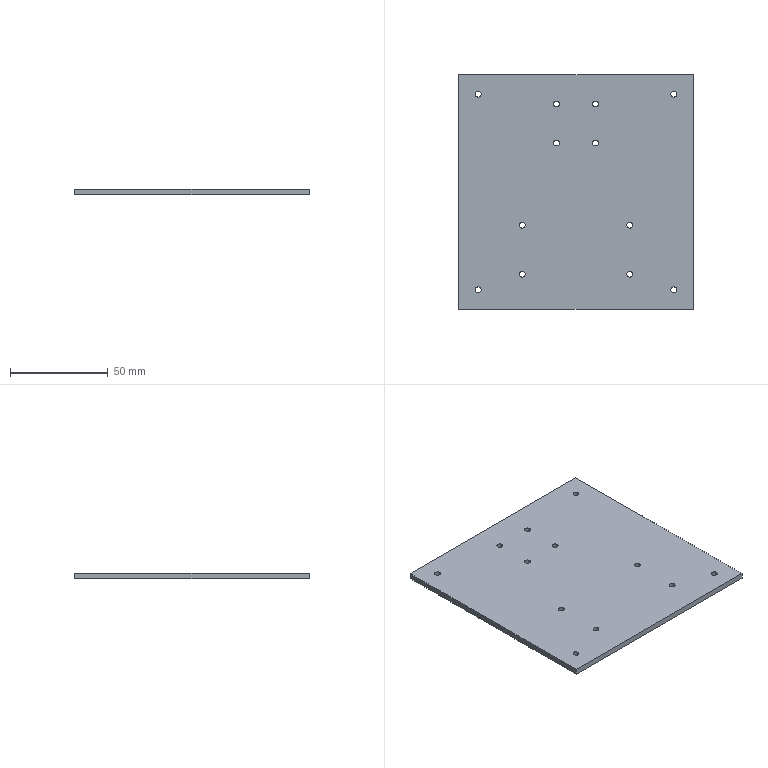Component | SolidWorks | Assembly3-1_Plate3-1 | 1 solid | 30 faces | box 120 x 120 x 3 mm | volume 42946 mm3 | cylinder 24 | plane 6 | commonest cylinder face diameters 3 x24
build123d program:
from build123d import *

# Parameters (mm, degrees)
SKETCH1_W           = 120
SKETCH1_H           = 120
BOSS_EXTRUDE1_DEPTH = 3
SKETCH2_R           = 1.5
CUT_EXTRUDE1_DEPTH  = 3
SKETCH5_R           = 1.5
CUT_EXTRUDE2_DEPTH  = 10


with BuildPart() as part:
    # Sketch1 → Boss-Extrude1 (new body)
    with BuildSketch(Plane.XY):
        Rectangle(SKETCH1_W, SKETCH1_H)
    extrude(amount=BOSS_EXTRUDE1_DEPTH)

    # Sketch2 → Cut-Extrude1 (cut)
    with BuildSketch(Plane.XY.offset(3)):
        with Locations((-50, 50)):
            Circle(SKETCH2_R)
        with Locations(Location((50, 50, 0), (0, 0, 180))):
            Circle(SKETCH2_R)
        with Locations((50, -50)):
            Circle(SKETCH2_R)
        with Locations(Location((-50, -50, 0), (0, 0, 180))):
            Circle(SKETCH2_R)
    extrude(amount=-CUT_EXTRUDE1_DEPTH, mode=Mode.SUBTRACT)

    # Sketch5 → Cut-Extrude2 (cut)
    with BuildSketch(Plane.XY.offset(3)):
        with Locations((-27.5, 42)):
            Circle(SKETCH5_R)
        with Locations((27.5, 42)):
            Circle(SKETCH5_R)
        with Locations((-10, -45)):
            Circle(SKETCH5_R)
        with Locations((10, -45)):
            Circle(SKETCH5_R)
        with Locations((-27.5, 17)):
            Circle(SKETCH5_R)
        with Locations((27.5, 17)):
            Circle(SKETCH5_R)
        with Locations((-10, -25)):
            Circle(SKETCH5_R)
        with Locations((10, -25)):
            Circle(SKETCH5_R)
    extrude(amount=-CUT_EXTRUDE2_DEPTH, mode=Mode.SUBTRACT)


solid = part.part

# Placed as in the assembly
solid = solid.moved(Location((0, 0, 52), (180, 0, 0)))
STEP:
#1=COLOUR_RGB('',0.7922,0.8196,0.9333);
#2=FILL_AREA_STYLE_COLOUR('',#1);
#3=FILL_AREA_STYLE('',(#2));
#4=SURFACE_STYLE_FILL_AREA(#3);
#5=SURFACE_SIDE_STYLE('',(#4));
#6=SURFACE_STYLE_USAGE(.BOTH.,#5);
#7=PRESENTATION_STYLE_ASSIGNMENT((#6));
#8=CARTESIAN_POINT('',(-1.142,-0.6693,2.047));
#9=VERTEX_POINT('',#8);
#10=CARTESIAN_POINT('',(-1.024,-0.6693,2.047));
#11=VERTEX_POINT('',#10);
#12=CARTESIAN_POINT('',(-1.083,-0.6693,2.047));
#13=DIRECTION('',(-0.,-0.,-1.));
#14=DIRECTION('',(1.,0.,0.));
#15=AXIS2_PLACEMENT_3D('',#12,#13,#14);
#16=CIRCLE('',#15,0.05906);
#17=EDGE_CURVE('',#9,#11,#16,.T.);
#18=ORIENTED_EDGE('',*,*,#17,.F.);
#19=CARTESIAN_POINT('',(-1.142,-0.6693,1.929));
#20=VERTEX_POINT('',#19);
#21=CARTESIAN_POINT('',(-1.142,-0.6693,2.323));
#22=DIRECTION('',(-0.,-0.,-1.));
#23=VECTOR('',#22,39.37);
#24=LINE('',#21,#23);
#25=EDGE_CURVE('',#9,#20,#24,.T.);
#26=ORIENTED_EDGE('',*,*,#25,.T.);
#27=CARTESIAN_POINT('',(-1.024,-0.6693,1.929));
#28=VERTEX_POINT('',#27);
#29=CARTESIAN_POINT('',(-1.083,-0.6693,1.929));
#30=DIRECTION('',(-0.,-0.,-1.));
#31=DIRECTION('',(1.,0.,0.));
#32=AXIS2_PLACEMENT_3D('',#29,#30,#31);
#33=CIRCLE('',#32,0.05906);
#34=EDGE_CURVE('',#20,#28,#33,.T.);
#35=ORIENTED_EDGE('',*,*,#34,.T.);
#36=CARTESIAN_POINT('',(-1.024,-0.6693,2.323));
#37=DIRECTION('',(-0.,-0.,-1.));
#38=VECTOR('',#37,39.37);
#39=LINE('',#36,#38);
#40=EDGE_CURVE('',#11,#28,#39,.T.);
#41=ORIENTED_EDGE('',*,*,#40,.F.);
#42=EDGE_LOOP('',(#18,#26,#35,#41));
#43=FACE_OUTER_BOUND('',#42,.T.);
#44=CARTESIAN_POINT('',(-1.083,-0.6693,2.323));
#45=DIRECTION('',(-0.,-0.,-1.));
#46=DIRECTION('',(1.,0.,0.));
#47=AXIS2_PLACEMENT_3D('',#44,#45,#46);
#48=CYLINDRICAL_SURFACE('',#47,0.05906);
#49=ADVANCED_FACE('',(#43),#48,.F.);
#50=CARTESIAN_POINT('',(0.3346,1.772,2.047));
#51=VERTEX_POINT('',#50);
#52=CARTESIAN_POINT('',(0.4528,1.772,2.047));
#53=VERTEX_POINT('',#52);
#54=CARTESIAN_POINT('',(0.3937,1.772,2.047));
#55=DIRECTION('',(-0.,-0.,-1.));
#56=DIRECTION('',(1.,0.,0.));
#57=AXIS2_PLACEMENT_3D('',#54,#55,#56);
#58=CIRCLE('',#57,0.05906);
#59=EDGE_CURVE('',#51,#53,#58,.T.);
#60=ORIENTED_EDGE('',*,*,#59,.F.);
#61=CARTESIAN_POINT('',(0.3346,1.772,1.929));
#62=VERTEX_POINT('',#61);
#63=CARTESIAN_POINT('',(0.3346,1.772,2.323));
#64=DIRECTION('',(-0.,-0.,-1.));
#65=VECTOR('',#64,39.37);
#66=LINE('',#63,#65);
#67=EDGE_CURVE('',#51,#62,#66,.T.);
#68=ORIENTED_EDGE('',*,*,#67,.T.);
#69=CARTESIAN_POINT('',(0.4528,1.772,1.929));
#70=VERTEX_POINT('',#69);
#71=CARTESIAN_POINT('',(0.3937,1.772,1.929));
#72=DIRECTION('',(-0.,-0.,-1.));
#73=DIRECTION('',(-1.,0.,0.));
#74=AXIS2_PLACEMENT_3D('',#71,#72,#73);
#75=CIRCLE('',#74,0.05906);
#76=EDGE_CURVE('',#62,#70,#75,.T.);
#77=ORIENTED_EDGE('',*,*,#76,.T.);
#78=CARTESIAN_POINT('',(0.4528,1.772,2.323));
#79=DIRECTION('',(-0.,-0.,-1.));
#80=VECTOR('',#79,39.37);
#81=LINE('',#78,#80);
#82=EDGE_CURVE('',#53,#70,#81,.T.);
#83=ORIENTED_EDGE('',*,*,#82,.F.);
#84=EDGE_LOOP('',(#60,#68,#77,#83));
#85=FACE_OUTER_BOUND('',#84,.T.);
#86=CARTESIAN_POINT('',(0.3937,1.772,2.323));
#87=DIRECTION('',(-0.,-0.,-1.));
#88=DIRECTION('',(1.,0.,0.));
#89=AXIS2_PLACEMENT_3D('',#86,#87,#88);
#90=CYLINDRICAL_SURFACE('',#89,0.05906);
#91=ADVANCED_FACE('',(#85),#90,.F.);
#92=CARTESIAN_POINT('',(-0.4528,1.772,2.047));
#93=VERTEX_POINT('',#92);
#94=CARTESIAN_POINT('',(-0.3346,1.772,2.047));
#95=VERTEX_POINT('',#94);
#96=CARTESIAN_POINT('',(-0.3937,1.772,2.047));
#97=DIRECTION('',(-0.,-0.,-1.));
#98=DIRECTION('',(1.,0.,0.));
#99=AXIS2_PLACEMENT_3D('',#96,#97,#98);
#100=CIRCLE('',#99,0.05906);
#101=EDGE_CURVE('',#93,#95,#100,.T.);
#102=ORIENTED_EDGE('',*,*,#101,.F.);
#103=CARTESIAN_POINT('',(-0.4528,1.772,1.929));
#104=VERTEX_POINT('',#103);
#105=CARTESIAN_POINT('',(-0.4528,1.772,2.323));
#106=DIRECTION('',(-0.,-0.,-1.));
#107=VECTOR('',#106,39.37);
#108=LINE('',#105,#107);
#109=EDGE_CURVE('',#93,#104,#108,.T.);
#110=ORIENTED_EDGE('',*,*,#109,.T.);
#111=CARTESIAN_POINT('',(-0.3346,1.772,1.929));
#112=VERTEX_POINT('',#111);
#113=CARTESIAN_POINT('',(-0.3937,1.772,1.929));
#114=DIRECTION('',(-0.,-0.,-1.));
#115=DIRECTION('',(1.,0.,0.));
#116=AXIS2_PLACEMENT_3D('',#113,#114,#115);
#117=CIRCLE('',#116,0.05906);
#118=EDGE_CURVE('',#104,#112,#117,.T.);
#119=ORIENTED_EDGE('',*,*,#118,.T.);
#120=CARTESIAN_POINT('',(-0.3346,1.772,2.323));
#121=DIRECTION('',(-0.,-0.,-1.));
#122=VECTOR('',#121,39.37);
#123=LINE('',#120,#122);
#124=EDGE_CURVE('',#95,#112,#123,.T.);
#125=ORIENTED_EDGE('',*,*,#124,.F.);
#126=EDGE_LOOP('',(#102,#110,#119,#125));
#127=FACE_OUTER_BOUND('',#126,.T.);
#128=CARTESIAN_POINT('',(-0.3937,1.772,2.323));
#129=DIRECTION('',(-0.,-0.,-1.));
#130=DIRECTION('',(1.,0.,0.));
#131=AXIS2_PLACEMENT_3D('',#128,#129,#130);
#132=CYLINDRICAL_SURFACE('',#131,0.05906);
#133=ADVANCED_FACE('',(#127),#132,.F.);
#134=CARTESIAN_POINT('',(1.024,-1.654,2.047));
#135=VERTEX_POINT('',#134);
#136=CARTESIAN_POINT('',(1.142,-1.654,2.047));
#137=VERTEX_POINT('',#136);
#138=CARTESIAN_POINT('',(1.083,-1.654,2.047));
#139=DIRECTION('',(-0.,-0.,-1.));
#140=DIRECTION('',(1.,0.,0.));
#141=AXIS2_PLACEMENT_3D('',#138,#139,#140);
#142=CIRCLE('',#141,0.05906);
#143=EDGE_CURVE('',#135,#137,#142,.T.);
#144=ORIENTED_EDGE('',*,*,#143,.F.);
#145=CARTESIAN_POINT('',(1.024,-1.654,1.929));
#146=VERTEX_POINT('',#145);
#147=CARTESIAN_POINT('',(1.024,-1.654,2.323));
#148=DIRECTION('',(-0.,-0.,-1.));
#149=VECTOR('',#148,39.37);
#150=LINE('',#147,#149);
#151=EDGE_CURVE('',#135,#146,#150,.T.);
#152=ORIENTED_EDGE('',*,*,#151,.T.);
#153=CARTESIAN_POINT('',(1.142,-1.654,1.929));
#154=VERTEX_POINT('',#153);
#155=CARTESIAN_POINT('',(1.083,-1.654,1.929));
#156=DIRECTION('',(-0.,-0.,-1.));
#157=DIRECTION('',(-1.,0.,0.));
#158=AXIS2_PLACEMENT_3D('',#155,#156,#157);
#159=CIRCLE('',#158,0.05906);
#160=EDGE_CURVE('',#146,#154,#159,.T.);
#161=ORIENTED_EDGE('',*,*,#160,.T.);
#162=CARTESIAN_POINT('',(1.142,-1.654,2.323));
#163=DIRECTION('',(-0.,-0.,-1.));
#164=VECTOR('',#163,39.37);
#165=LINE('',#162,#164);
#166=EDGE_CURVE('',#137,#154,#165,.T.);
#167=ORIENTED_EDGE('',*,*,#166,.F.);
#168=EDGE_LOOP('',(#144,#152,#161,#167));
#169=FACE_OUTER_BOUND('',#168,.T.);
#170=CARTESIAN_POINT('',(1.083,-1.654,2.323));
#171=DIRECTION('',(-0.,-0.,-1.));
#172=DIRECTION('',(1.,0.,0.));
#173=AXIS2_PLACEMENT_3D('',#170,#171,#172);
#174=CYLINDRICAL_SURFACE('',#173,0.05906);
#175=ADVANCED_FACE('',(#169),#174,.F.);
#176=CARTESIAN_POINT('',(0.3346,0.9843,2.047));
#177=VERTEX_POINT('',#176);
#178=CARTESIAN_POINT('',(0.4528,0.9843,2.047));
#179=VERTEX_POINT('',#178);
#180=CARTESIAN_POINT('',(0.3937,0.9843,2.047));
#181=DIRECTION('',(-0.,-0.,-1.));
#182=DIRECTION('',(1.,0.,0.));
#183=AXIS2_PLACEMENT_3D('',#180,#181,#182);
#184=CIRCLE('',#183,0.05906);
#185=EDGE_CURVE('',#177,#179,#184,.T.);
#186=ORIENTED_EDGE('',*,*,#185,.F.);
#187=CARTESIAN_POINT('',(0.3346,0.9843,1.929));
#188=VERTEX_POINT('',#187);
#189=CARTESIAN_POINT('',(0.3346,0.9843,2.323));
#190=DIRECTION('',(-0.,-0.,-1.));
#191=VECTOR('',#190,39.37);
#192=LINE('',#189,#191);
#193=EDGE_CURVE('',#177,#188,#192,.T.);
#194=ORIENTED_EDGE('',*,*,#193,.T.);
#195=CARTESIAN_POINT('',(0.4528,0.9843,1.929));
#196=VERTEX_POINT('',#195);
#197=CARTESIAN_POINT('',(0.3937,0.9843,1.929));
#198=DIRECTION('',(-0.,-0.,-1.));
#199=DIRECTION('',(1.,0.,0.));
#200=AXIS2_PLACEMENT_3D('',#197,#198,#199);
#201=CIRCLE('',#200,0.05906);
#202=EDGE_CURVE('',#188,#196,#201,.T.);
#203=ORIENTED_EDGE('',*,*,#202,.T.);
#204=CARTESIAN_POINT('',(0.4528,0.9843,2.323));
#205=DIRECTION('',(-0.,-0.,-1.));
#206=VECTOR('',#205,39.37);
#207=LINE('',#204,#206);
#208=EDGE_CURVE('',#179,#196,#207,.T.);
#209=ORIENTED_EDGE('',*,*,#208,.F.);
#210=EDGE_LOOP('',(#186,#194,#203,#209));
#211=FACE_OUTER_BOUND('',#210,.T.);
#212=CARTESIAN_POINT('',(0.3937,0.9843,2.323));
#213=DIRECTION('',(-0.,-0.,-1.));
#214=DIRECTION('',(1.,0.,0.));
#215=AXIS2_PLACEMENT_3D('',#212,#213,#214);
#216=CYLINDRICAL_SURFACE('',#215,0.05906);
#217=ADVANCED_FACE('',(#211),#216,.F.);
#218=CARTESIAN_POINT('',(-0.4528,0.9843,2.047));
#219=VERTEX_POINT('',#218);
#220=CARTESIAN_POINT('',(-0.3346,0.9843,2.047));
#221=VERTEX_POINT('',#220);
#222=CARTESIAN_POINT('',(-0.3937,0.9843,2.047));
#223=DIRECTION('',(-0.,-0.,-1.));
#224=DIRECTION('',(1.,0.,0.));
#225=AXIS2_PLACEMENT_3D('',#222,#223,#224);
#226=CIRCLE('',#225,0.05906);
#227=EDGE_CURVE('',#219,#221,#226,.T.);
#228=ORIENTED_EDGE('',*,*,#227,.F.);
#229=CARTESIAN_POINT('',(-0.4528,0.9843,1.929));
#230=VERTEX_POINT('',#229);
#231=CARTESIAN_POINT('',(-0.4528,0.9843,2.323));
#232=DIRECTION('',(-0.,-0.,-1.));
#233=VECTOR('',#232,39.37);
#234=LINE('',#231,#233);
#235=EDGE_CURVE('',#219,#230,#234,.T.);
#236=ORIENTED_EDGE('',*,*,#235,.T.);
#237=CARTESIAN_POINT('',(-0.3346,0.9843,1.929));
#238=VERTEX_POINT('',#237);
#239=CARTESIAN_POINT('',(-0.3937,0.9843,1.929));
#240=DIRECTION('',(-0.,-0.,-1.));
#241=DIRECTION('',(1.,0.,0.));
#242=AXIS2_PLACEMENT_3D('',#239,#240,#241);
#243=CIRCLE('',#242,0.05906);
#244=EDGE_CURVE('',#230,#238,#243,.T.);
#245=ORIENTED_EDGE('',*,*,#244,.T.);
#246=CARTESIAN_POINT('',(-0.3346,0.9843,2.323));
#247=DIRECTION('',(-0.,-0.,-1.));
#248=VECTOR('',#247,39.37);
#249=LINE('',#246,#248);
#250=EDGE_CURVE('',#221,#238,#249,.T.);
#251=ORIENTED_EDGE('',*,*,#250,.F.);
#252=EDGE_LOOP('',(#228,#236,#245,#251));
#253=FACE_OUTER_BOUND('',#252,.T.);
#254=CARTESIAN_POINT('',(-0.3937,0.9843,2.323));
#255=DIRECTION('',(-0.,-0.,-1.));
#256=DIRECTION('',(1.,0.,0.));
#257=AXIS2_PLACEMENT_3D('',#254,#255,#256);
#258=CYLINDRICAL_SURFACE('',#257,0.05906);
#259=ADVANCED_FACE('',(#253),#258,.F.);
#260=CARTESIAN_POINT('',(1.024,-0.6693,2.047));
#261=VERTEX_POINT('',#260);
#262=CARTESIAN_POINT('',(1.142,-0.6693,2.047));
#263=VERTEX_POINT('',#262);
#264=CARTESIAN_POINT('',(1.083,-0.6693,2.047));
#265=DIRECTION('',(-0.,-0.,-1.));
#266=DIRECTION('',(1.,0.,0.));
#267=AXIS2_PLACEMENT_3D('',#264,#265,#266);
#268=CIRCLE('',#267,0.05906);
#269=EDGE_CURVE('',#261,#263,#268,.T.);
#270=ORIENTED_EDGE('',*,*,#269,.F.);
#271=CARTESIAN_POINT('',(1.024,-0.6693,1.929));
#272=VERTEX_POINT('',#271);
#273=CARTESIAN_POINT('',(1.024,-0.6693,2.323));
#274=DIRECTION('',(-0.,-0.,-1.));
#275=VECTOR('',#274,39.37);
#276=LINE('',#273,#275);
#277=EDGE_CURVE('',#261,#272,#276,.T.);
#278=ORIENTED_EDGE('',*,*,#277,.T.);
#279=CARTESIAN_POINT('',(1.142,-0.6693,1.929));
#280=VERTEX_POINT('',#279);
#281=CARTESIAN_POINT('',(1.083,-0.6693,1.929));
#282=DIRECTION('',(-0.,-0.,-1.));
#283=DIRECTION('',(-1.,0.,0.));
#284=AXIS2_PLACEMENT_3D('',#281,#282,#283);
#285=CIRCLE('',#284,0.05906);
#286=EDGE_CURVE('',#272,#280,#285,.T.);
#287=ORIENTED_EDGE('',*,*,#286,.T.);
#288=CARTESIAN_POINT('',(1.142,-0.6693,2.323));
#289=DIRECTION('',(-0.,-0.,-1.));
#290=VECTOR('',#289,39.37);
#291=LINE('',#288,#290);
#292=EDGE_CURVE('',#263,#280,#291,.T.);
#293=ORIENTED_EDGE('',*,*,#292,.F.);
#294=EDGE_LOOP('',(#270,#278,#287,#293));
#295=FACE_OUTER_BOUND('',#294,.T.);
#296=CARTESIAN_POINT('',(1.083,-0.6693,2.323));
#297=DIRECTION('',(-0.,-0.,-1.));
#298=DIRECTION('',(1.,0.,0.));
#299=AXIS2_PLACEMENT_3D('',#296,#297,#298);
#300=CYLINDRICAL_SURFACE('',#299,0.05906);
#301=ADVANCED_FACE('',(#295),#300,.F.);
#302=CARTESIAN_POINT('',(-1.142,-1.654,2.047));
#303=VERTEX_POINT('',#302);
#304=CARTESIAN_POINT('',(-1.024,-1.654,2.047));
#305=VERTEX_POINT('',#304);
#306=CARTESIAN_POINT('',(-1.083,-1.654,2.047));
#307=DIRECTION('',(-0.,-0.,-1.));
#308=DIRECTION('',(1.,0.,0.));
#309=AXIS2_PLACEMENT_3D('',#306,#307,#308);
#310=CIRCLE('',#309,0.05906);
#311=EDGE_CURVE('',#303,#305,#310,.T.);
#312=ORIENTED_EDGE('',*,*,#311,.F.);
#313=CARTESIAN_POINT('',(-1.142,-1.654,1.929));
#314=VERTEX_POINT('',#313);
#315=CARTESIAN_POINT('',(-1.142,-1.654,2.323));
#316=DIRECTION('',(-0.,-0.,-1.));
#317=VECTOR('',#316,39.37);
#318=LINE('',#315,#317);
#319=EDGE_CURVE('',#303,#314,#318,.T.);
#320=ORIENTED_EDGE('',*,*,#319,.T.);
#321=CARTESIAN_POINT('',(-1.024,-1.654,1.929));
#322=VERTEX_POINT('',#321);
#323=CARTESIAN_POINT('',(-1.083,-1.654,1.929));
#324=DIRECTION('',(-0.,-0.,-1.));
#325=DIRECTION('',(1.,0.,0.));
#326=AXIS2_PLACEMENT_3D('',#323,#324,#325);
#327=CIRCLE('',#326,0.05906);
#328=EDGE_CURVE('',#314,#322,#327,.T.);
#329=ORIENTED_EDGE('',*,*,#328,.T.);
#330=CARTESIAN_POINT('',(-1.024,-1.654,2.323));
#331=DIRECTION('',(-0.,-0.,-1.));
#332=VECTOR('',#331,39.37);
#333=LINE('',#330,#332);
#334=EDGE_CURVE('',#305,#322,#333,.T.);
#335=ORIENTED_EDGE('',*,*,#334,.F.);
#336=EDGE_LOOP('',(#312,#320,#329,#335));
#337=FACE_OUTER_BOUND('',#336,.T.);
#338=CARTESIAN_POINT('',(-1.083,-1.654,2.323));
#339=DIRECTION('',(-0.,-0.,-1.));
#340=DIRECTION('',(1.,0.,0.));
#341=AXIS2_PLACEMENT_3D('',#338,#339,#340);
#342=CYLINDRICAL_SURFACE('',#341,0.05906);
#343=ADVANCED_FACE('',(#337),#342,.F.);
#344=CARTESIAN_POINT('',(-2.028,1.969,2.047));
#345=VERTEX_POINT('',#344);
#346=CARTESIAN_POINT('',(-1.909,1.969,2.047));
#347=VERTEX_POINT('',#346);
#348=CARTESIAN_POINT('',(-1.969,1.969,2.047));
#349=DIRECTION('',(-0.,-0.,-1.));
#350=DIRECTION('',(-1.,0.,0.));
#351=AXIS2_PLACEMENT_3D('',#348,#349,#350);
#352=CIRCLE('',#351,0.05906);
#353=EDGE_CURVE('',#345,#347,#352,.T.);
#354=ORIENTED_EDGE('',*,*,#353,.F.);
#355=CARTESIAN_POINT('',(-2.028,1.969,1.929));
#356=VERTEX_POINT('',#355);
#357=CARTESIAN_POINT('',(-2.028,1.969,2.047));
#358=DIRECTION('',(-0.,-0.,-1.));
#359=VECTOR('',#358,39.37);
#360=LINE('',#357,#359);
#361=EDGE_CURVE('',#345,#356,#360,.T.);
#362=ORIENTED_EDGE('',*,*,#361,.T.);
#363=CARTESIAN_POINT('',(-1.909,1.969,1.929));
#364=VERTEX_POINT('',#363);
#365=CARTESIAN_POINT('',(-1.969,1.969,1.929));
#366=DIRECTION('',(-0.,-0.,-1.));
#367=DIRECTION('',(-1.,0.,0.));
#368=AXIS2_PLACEMENT_3D('',#365,#366,#367);
#369=CIRCLE('',#368,0.05906);
#370=EDGE_CURVE('',#356,#364,#369,.T.);
#371=ORIENTED_EDGE('',*,*,#370,.T.);
#372=CARTESIAN_POINT('',(-1.909,1.969,2.047));
#373=DIRECTION('',(-0.,-0.,-1.));
#374=VECTOR('',#373,39.37);
#375=LINE('',#372,#374);
#376=EDGE_CURVE('',#347,#364,#375,.T.);
#377=ORIENTED_EDGE('',*,*,#376,.F.);
#378=EDGE_LOOP('',(#354,#362,#371,#377));
#379=FACE_OUTER_BOUND('',#378,.T.);
#380=CARTESIAN_POINT('',(-1.969,1.969,2.047));
#381=DIRECTION('',(-0.,-0.,-1.));
#382=DIRECTION('',(1.,0.,0.));
#383=AXIS2_PLACEMENT_3D('',#380,#381,#382);
#384=CYLINDRICAL_SURFACE('',#383,0.05906);
#385=ADVANCED_FACE('',(#379),#384,.F.);
#386=CARTESIAN_POINT('',(1.909,1.969,2.047));
#387=VERTEX_POINT('',#386);
#388=CARTESIAN_POINT('',(2.028,1.969,2.047));
#389=VERTEX_POINT('',#388);
#390=CARTESIAN_POINT('',(1.969,1.969,2.047));
#391=DIRECTION('',(-0.,-0.,-1.));
#392=DIRECTION('',(1.,0.,0.));
#393=AXIS2_PLACEMENT_3D('',#390,#391,#392);
#394=CIRCLE('',#393,0.05906);
#395=EDGE_CURVE('',#387,#389,#394,.T.);
#396=ORIENTED_EDGE('',*,*,#395,.F.);
#397=CARTESIAN_POINT('',(1.909,1.969,1.929));
#398=VERTEX_POINT('',#397);
#399=CARTESIAN_POINT('',(1.909,1.969,2.047));
#400=DIRECTION('',(-0.,-0.,-1.));
#401=VECTOR('',#400,39.37);
#402=LINE('',#399,#401);
#403=EDGE_CURVE('',#387,#398,#402,.T.);
#404=ORIENTED_EDGE('',*,*,#403,.T.);
#405=CARTESIAN_POINT('',(2.028,1.969,1.929));
#406=VERTEX_POINT('',#405);
#407=CARTESIAN_POINT('',(1.969,1.969,1.929));
#408=DIRECTION('',(-0.,-0.,-1.));
#409=DIRECTION('',(1.,0.,0.));
#410=AXIS2_PLACEMENT_3D('',#407,#408,#409);
#411=CIRCLE('',#410,0.05906);
#412=EDGE_CURVE('',#398,#406,#411,.T.);
#413=ORIENTED_EDGE('',*,*,#412,.T.);
#414=CARTESIAN_POINT('',(2.028,1.969,2.047));
#415=DIRECTION('',(-0.,-0.,-1.));
#416=VECTOR('',#415,39.37);
#417=LINE('',#414,#416);
#418=EDGE_CURVE('',#389,#406,#417,.T.);
#419=ORIENTED_EDGE('',*,*,#418,.F.);
#420=EDGE_LOOP('',(#396,#404,#413,#419));
#421=FACE_OUTER_BOUND('',#420,.T.);
#422=CARTESIAN_POINT('',(1.969,1.969,2.047));
#423=DIRECTION('',(-0.,-0.,-1.));
#424=DIRECTION('',(1.,0.,0.));
#425=AXIS2_PLACEMENT_3D('',#422,#423,#424);
#426=CYLINDRICAL_SURFACE('',#425,0.05906);
#427=ADVANCED_FACE('',(#421),#426,.F.);
#428=CARTESIAN_POINT('',(1.909,-1.969,2.047));
#429=VERTEX_POINT('',#428);
#430=CARTESIAN_POINT('',(2.028,-1.969,2.047));
#431=VERTEX_POINT('',#430);
#432=CARTESIAN_POINT('',(1.969,-1.969,2.047));
#433=DIRECTION('',(-0.,-0.,-1.));
#434=DIRECTION('',(-1.,0.,0.));
#435=AXIS2_PLACEMENT_3D('',#432,#433,#434);
#436=CIRCLE('',#435,0.05906);
#437=EDGE_CURVE('',#429,#431,#436,.T.);
#438=ORIENTED_EDGE('',*,*,#437,.F.);
#439=CARTESIAN_POINT('',(1.909,-1.969,1.929));
#440=VERTEX_POINT('',#439);
#441=CARTESIAN_POINT('',(1.909,-1.969,2.047));
#442=DIRECTION('',(-0.,-0.,-1.));
#443=VECTOR('',#442,39.37);
#444=LINE('',#441,#443);
#445=EDGE_CURVE('',#429,#440,#444,.T.);
#446=ORIENTED_EDGE('',*,*,#445,.T.);
#447=CARTESIAN_POINT('',(2.028,-1.969,1.929));
#448=VERTEX_POINT('',#447);
#449=CARTESIAN_POINT('',(1.969,-1.969,1.929));
#450=DIRECTION('',(-0.,-0.,-1.));
#451=DIRECTION('',(-1.,0.,0.));
#452=AXIS2_PLACEMENT_3D('',#449,#450,#451);
#453=CIRCLE('',#452,0.05906);
#454=EDGE_CURVE('',#440,#448,#453,.T.);
#455=ORIENTED_EDGE('',*,*,#454,.T.);
#456=CARTESIAN_POINT('',(2.028,-1.969,2.047));
#457=DIRECTION('',(-0.,-0.,-1.));
#458=VECTOR('',#457,39.37);
#459=LINE('',#456,#458);
#460=EDGE_CURVE('',#431,#448,#459,.T.);
#461=ORIENTED_EDGE('',*,*,#460,.F.);
#462=EDGE_LOOP('',(#438,#446,#455,#461));
#463=FACE_OUTER_BOUND('',#462,.T.);
#464=CARTESIAN_POINT('',(1.969,-1.969,2.047));
#465=DIRECTION('',(-0.,-0.,-1.));
#466=DIRECTION('',(1.,0.,0.));
#467=AXIS2_PLACEMENT_3D('',#464,#465,#466);
#468=CYLINDRICAL_SURFACE('',#467,0.05906);
#469=ADVANCED_FACE('',(#463),#468,.F.);
#470=CARTESIAN_POINT('',(-2.028,-1.969,2.047));
#471=VERTEX_POINT('',#470);
#472=CARTESIAN_POINT('',(-1.909,-1.969,2.047));
#473=VERTEX_POINT('',#472);
#474=CARTESIAN_POINT('',(-1.969,-1.969,2.047));
#475=DIRECTION('',(-0.,-0.,-1.));
#476=DIRECTION('',(1.,0.,0.));
#477=AXIS2_PLACEMENT_3D('',#474,#475,#476);
#478=CIRCLE('',#477,0.05906);
#479=EDGE_CURVE('',#471,#473,#478,.T.);
#480=ORIENTED_EDGE('',*,*,#479,.F.);
#481=CARTESIAN_POINT('',(-2.028,-1.969,1.929));
#482=VERTEX_POINT('',#481);
#483=CARTESIAN_POINT('',(-2.028,-1.969,2.047));
#484=DIRECTION('',(-0.,-0.,-1.));
#485=VECTOR('',#484,39.37);
#486=LINE('',#483,#485);
#487=EDGE_CURVE('',#471,#482,#486,.T.);
#488=ORIENTED_EDGE('',*,*,#487,.T.);
#489=CARTESIAN_POINT('',(-1.909,-1.969,1.929));
#490=VERTEX_POINT('',#489);
#491=CARTESIAN_POINT('',(-1.969,-1.969,1.929));
#492=DIRECTION('',(-0.,-0.,-1.));
#493=DIRECTION('',(1.,0.,0.));
#494=AXIS2_PLACEMENT_3D('',#491,#492,#493);
#495=CIRCLE('',#494,0.05906);
#496=EDGE_CURVE('',#482,#490,#495,.T.);
#497=ORIENTED_EDGE('',*,*,#496,.T.);
#498=CARTESIAN_POINT('',(-1.909,-1.969,2.047));
#499=DIRECTION('',(-0.,-0.,-1.));
#500=VECTOR('',#499,39.37);
#501=LINE('',#498,#500);
#502=EDGE_CURVE('',#473,#490,#501,.T.);
#503=ORIENTED_EDGE('',*,*,#502,.F.);
#504=EDGE_LOOP('',(#480,#488,#497,#503));
#505=FACE_OUTER_BOUND('',#504,.T.);
#506=CARTESIAN_POINT('',(-1.969,-1.969,2.047));
#507=DIRECTION('',(-0.,-0.,-1.));
#508=DIRECTION('',(1.,0.,0.));
#509=AXIS2_PLACEMENT_3D('',#506,#507,#508);
#510=CYLINDRICAL_SURFACE('',#509,0.05906);
#511=ADVANCED_FACE('',(#505),#510,.F.);
#512=CARTESIAN_POINT('',(2.362,2.362,2.047));
#513=VERTEX_POINT('',#512);
#514=CARTESIAN_POINT('',(2.362,-2.362,2.047));
#515=VERTEX_POINT('',#514);
#516=CARTESIAN_POINT('',(2.362,-2.362,2.047));
#517=DIRECTION('',(0.,-1.,0.));
#518=VECTOR('',#517,39.37);
#519=LINE('',#516,#518);
#520=EDGE_CURVE('',#513,#515,#519,.T.);
#521=ORIENTED_EDGE('',*,*,#520,.T.);
#522=CARTESIAN_POINT('',(2.362,-2.362,1.929));
#523=VERTEX_POINT('',#522);
#524=CARTESIAN_POINT('',(2.362,-2.362,1.929));
#525=DIRECTION('',(0.,0.,1.));
#526=VECTOR('',#525,39.37);
#527=LINE('',#524,#526);
#528=EDGE_CURVE('',#523,#515,#527,.T.);
#529=ORIENTED_EDGE('',*,*,#528,.F.);
#530=CARTESIAN_POINT('',(2.362,2.362,1.929));
#531=VERTEX_POINT('',#530);
#532=CARTESIAN_POINT('',(2.362,-2.362,1.929));
#533=DIRECTION('',(0.,-1.,0.));
#534=VECTOR('',#533,39.37);
#535=LINE('',#532,#534);
#536=EDGE_CURVE('',#531,#523,#535,.T.);
#537=ORIENTED_EDGE('',*,*,#536,.F.);
#538=CARTESIAN_POINT('',(2.362,2.362,1.929));
#539=DIRECTION('',(0.,0.,1.));
#540=VECTOR('',#539,39.37);
#541=LINE('',#538,#540);
#542=EDGE_CURVE('',#531,#513,#541,.T.);
#543=ORIENTED_EDGE('',*,*,#542,.T.);
#544=EDGE_LOOP('',(#521,#529,#537,#543));
#545=FACE_OUTER_BOUND('',#544,.T.);
#546=CARTESIAN_POINT('',(2.362,-2.362,1.929));
#547=DIRECTION('',(-1.,-0.,0.));
#548=DIRECTION('',(-0.,1.,-0.));
#549=AXIS2_PLACEMENT_3D('',#546,#547,#548);
#550=PLANE('',#549);
#551=ADVANCED_FACE('',(#545),#550,.F.);
#552=CARTESIAN_POINT('',(-2.362,-2.362,2.047));
#553=VERTEX_POINT('',#552);
#554=CARTESIAN_POINT('',(-2.362,-2.362,2.047));
#555=DIRECTION('',(-1.,-0.,0.));
#556=VECTOR('',#555,39.37);
#557=LINE('',#554,#556);
#558=EDGE_CURVE('',#515,#553,#557,.T.);
#559=ORIENTED_EDGE('',*,*,#558,.T.);
#560=CARTESIAN_POINT('',(-2.362,-2.362,1.929));
#561=VERTEX_POINT('',#560);
#562=CARTESIAN_POINT('',(-2.362,-2.362,1.929));
#563=DIRECTION('',(0.,0.,1.));
#564=VECTOR('',#563,39.37);
#565=LINE('',#562,#564);
#566=EDGE_CURVE('',#561,#553,#565,.T.);
#567=ORIENTED_EDGE('',*,*,#566,.F.);
#568=CARTESIAN_POINT('',(-2.362,-2.362,1.929));
#569=DIRECTION('',(-1.,-0.,0.));
#570=VECTOR('',#569,39.37);
#571=LINE('',#568,#570);
#572=EDGE_CURVE('',#523,#561,#571,.T.);
#573=ORIENTED_EDGE('',*,*,#572,.F.);
#574=ORIENTED_EDGE('',*,*,#528,.T.);
#575=EDGE_LOOP('',(#559,#567,#573,#574));
#576=FACE_OUTER_BOUND('',#575,.T.);
#577=CARTESIAN_POINT('',(-2.362,-2.362,1.929));
#578=DIRECTION('',(-0.,1.,-0.));
#579=DIRECTION('',(0.,0.,1.));
#580=AXIS2_PLACEMENT_3D('',#577,#578,#579);
#581=PLANE('',#580);
#582=ADVANCED_FACE('',(#576),#581,.F.);
#583=CARTESIAN_POINT('',(-2.362,2.362,2.047));
#584=VERTEX_POINT('',#583);
#585=CARTESIAN_POINT('',(-2.362,-2.362,2.047));
#586=DIRECTION('',(-0.,1.,-0.));
#587=VECTOR('',#586,39.37);
#588=LINE('',#585,#587);
#589=EDGE_CURVE('',#553,#584,#588,.T.);
#590=ORIENTED_EDGE('',*,*,#589,.T.);
#591=CARTESIAN_POINT('',(-2.362,2.362,1.929));
#592=VERTEX_POINT('',#591);
#593=CARTESIAN_POINT('',(-2.362,2.362,1.929));
#594=DIRECTION('',(0.,0.,1.));
#595=VECTOR('',#594,39.37);
#596=LINE('',#593,#595);
#597=EDGE_CURVE('',#592,#584,#596,.T.);
#598=ORIENTED_EDGE('',*,*,#597,.F.);
#599=CARTESIAN_POINT('',(-2.362,-2.362,1.929));
#600=DIRECTION('',(-0.,1.,-0.));
#601=VECTOR('',#600,39.37);
#602=LINE('',#599,#601);
#603=EDGE_CURVE('',#561,#592,#602,.T.);
#604=ORIENTED_EDGE('',*,*,#603,.F.);
#605=ORIENTED_EDGE('',*,*,#566,.T.);
#606=EDGE_LOOP('',(#590,#598,#604,#605));
#607=FACE_OUTER_BOUND('',#606,.T.);
#608=CARTESIAN_POINT('',(-2.362,-2.362,1.929));
#609=DIRECTION('',(1.,0.,-0.));
#610=DIRECTION('',(0.,-1.,0.));
#611=AXIS2_PLACEMENT_3D('',#608,#609,#610);
#612=PLANE('',#611);
#613=ADVANCED_FACE('',(#607),#612,.F.);
#614=CARTESIAN_POINT('',(-2.362,2.362,2.047));
#615=DIRECTION('',(1.,0.,-0.));
#616=VECTOR('',#615,39.37);
#617=LINE('',#614,#616);
#618=EDGE_CURVE('',#584,#513,#617,.T.);
#619=ORIENTED_EDGE('',*,*,#618,.T.);
#620=ORIENTED_EDGE('',*,*,#542,.F.);
#621=CARTESIAN_POINT('',(-2.362,2.362,1.929));
#622=DIRECTION('',(1.,0.,-0.));
#623=VECTOR('',#622,39.37);
#624=LINE('',#621,#623);
#625=EDGE_CURVE('',#592,#531,#624,.T.);
#626=ORIENTED_EDGE('',*,*,#625,.F.);
#627=ORIENTED_EDGE('',*,*,#597,.T.);
#628=EDGE_LOOP('',(#619,#620,#626,#627));
#629=FACE_OUTER_BOUND('',#628,.T.);
#630=CARTESIAN_POINT('',(-2.362,2.362,1.929));
#631=DIRECTION('',(0.,-1.,0.));
#632=DIRECTION('',(-0.,-0.,-1.));
#633=AXIS2_PLACEMENT_3D('',#630,#631,#632);
#634=PLANE('',#633);
#635=ADVANCED_FACE('',(#629),#634,.F.);
#636=CARTESIAN_POINT('',(-1.083,-0.6693,1.929));
#637=DIRECTION('',(-0.,-0.,-1.));
#638=DIRECTION('',(1.,0.,0.));
#639=AXIS2_PLACEMENT_3D('',#636,#637,#638);
#640=CIRCLE('',#639,0.05906);
#641=EDGE_CURVE('',#28,#20,#640,.T.);
#642=ORIENTED_EDGE('',*,*,#641,.F.);
#643=ORIENTED_EDGE('',*,*,#34,.F.);
#644=EDGE_LOOP('',(#642,#643));
#645=FACE_BOUND('',#644,.T.);
#646=CARTESIAN_POINT('',(0.3937,1.772,1.929));
#647=DIRECTION('',(-0.,-0.,-1.));
#648=DIRECTION('',(-1.,0.,0.));
#649=AXIS2_PLACEMENT_3D('',#646,#647,#648);
#650=CIRCLE('',#649,0.05906);
#651=EDGE_CURVE('',#70,#62,#650,.T.);
#652=ORIENTED_EDGE('',*,*,#651,.F.);
#653=ORIENTED_EDGE('',*,*,#76,.F.);
#654=EDGE_LOOP('',(#652,#653));
#655=FACE_BOUND('',#654,.T.);
#656=CARTESIAN_POINT('',(-0.3937,1.772,1.929));
#657=DIRECTION('',(-0.,-0.,-1.));
#658=DIRECTION('',(1.,0.,0.));
#659=AXIS2_PLACEMENT_3D('',#656,#657,#658);
#660=CIRCLE('',#659,0.05906);
#661=EDGE_CURVE('',#112,#104,#660,.T.);
#662=ORIENTED_EDGE('',*,*,#661,.F.);
#663=ORIENTED_EDGE('',*,*,#118,.F.);
#664=EDGE_LOOP('',(#662,#663));
#665=FACE_BOUND('',#664,.T.);
#666=CARTESIAN_POINT('',(1.083,-1.654,1.929));
#667=DIRECTION('',(-0.,-0.,-1.));
#668=DIRECTION('',(-1.,0.,0.));
#669=AXIS2_PLACEMENT_3D('',#666,#667,#668);
#670=CIRCLE('',#669,0.05906);
#671=EDGE_CURVE('',#154,#146,#670,.T.);
#672=ORIENTED_EDGE('',*,*,#671,.F.);
#673=ORIENTED_EDGE('',*,*,#160,.F.);
#674=EDGE_LOOP('',(#672,#673));
#675=FACE_BOUND('',#674,.T.);
#676=CARTESIAN_POINT('',(0.3937,0.9843,1.929));
#677=DIRECTION('',(-0.,-0.,-1.));
#678=DIRECTION('',(1.,0.,0.));
#679=AXIS2_PLACEMENT_3D('',#676,#677,#678);
#680=CIRCLE('',#679,0.05906);
#681=EDGE_CURVE('',#196,#188,#680,.T.);
#682=ORIENTED_EDGE('',*,*,#681,.F.);
#683=ORIENTED_EDGE('',*,*,#202,.F.);
#684=EDGE_LOOP('',(#682,#683));
#685=FACE_BOUND('',#684,.T.);
#686=CARTESIAN_POINT('',(-0.3937,0.9843,1.929));
#687=DIRECTION('',(-0.,-0.,-1.));
#688=DIRECTION('',(1.,0.,0.));
#689=AXIS2_PLACEMENT_3D('',#686,#687,#688);
#690=CIRCLE('',#689,0.05906);
#691=EDGE_CURVE('',#238,#230,#690,.T.);
#692=ORIENTED_EDGE('',*,*,#691,.F.);
#693=ORIENTED_EDGE('',*,*,#244,.F.);
#694=EDGE_LOOP('',(#692,#693));
#695=FACE_BOUND('',#694,.T.);
#696=CARTESIAN_POINT('',(1.083,-0.6693,1.929));
#697=DIRECTION('',(-0.,-0.,-1.));
#698=DIRECTION('',(-1.,0.,0.));
#699=AXIS2_PLACEMENT_3D('',#696,#697,#698);
#700=CIRCLE('',#699,0.05906);
#701=EDGE_CURVE('',#280,#272,#700,.T.);
#702=ORIENTED_EDGE('',*,*,#701,.F.);
#703=ORIENTED_EDGE('',*,*,#286,.F.);
#704=EDGE_LOOP('',(#702,#703));
#705=FACE_BOUND('',#704,.T.);
#706=CARTESIAN_POINT('',(-1.083,-1.654,1.929));
#707=DIRECTION('',(-0.,-0.,-1.));
#708=DIRECTION('',(1.,0.,0.));
#709=AXIS2_PLACEMENT_3D('',#706,#707,#708);
#710=CIRCLE('',#709,0.05906);
#711=EDGE_CURVE('',#322,#314,#710,.T.);
#712=ORIENTED_EDGE('',*,*,#711,.F.);
#713=ORIENTED_EDGE('',*,*,#328,.F.);
#714=EDGE_LOOP('',(#712,#713));
#715=FACE_BOUND('',#714,.T.);
#716=CARTESIAN_POINT('',(-1.969,1.969,1.929));
#717=DIRECTION('',(-0.,-0.,-1.));
#718=DIRECTION('',(-1.,0.,0.));
#719=AXIS2_PLACEMENT_3D('',#716,#717,#718);
#720=CIRCLE('',#719,0.05906);
#721=EDGE_CURVE('',#364,#356,#720,.T.);
#722=ORIENTED_EDGE('',*,*,#721,.F.);
#723=ORIENTED_EDGE('',*,*,#370,.F.);
#724=EDGE_LOOP('',(#722,#723));
#725=FACE_BOUND('',#724,.T.);
#726=CARTESIAN_POINT('',(1.969,1.969,1.929));
#727=DIRECTION('',(-0.,-0.,-1.));
#728=DIRECTION('',(1.,0.,0.));
#729=AXIS2_PLACEMENT_3D('',#726,#727,#728);
#730=CIRCLE('',#729,0.05906);
#731=EDGE_CURVE('',#406,#398,#730,.T.);
#732=ORIENTED_EDGE('',*,*,#731,.F.);
#733=ORIENTED_EDGE('',*,*,#412,.F.);
#734=EDGE_LOOP('',(#732,#733));
#735=FACE_BOUND('',#734,.T.);
#736=CARTESIAN_POINT('',(1.969,-1.969,1.929));
#737=DIRECTION('',(-0.,-0.,-1.));
#738=DIRECTION('',(-1.,0.,0.));
#739=AXIS2_PLACEMENT_3D('',#736,#737,#738);
#740=CIRCLE('',#739,0.05906);
#741=EDGE_CURVE('',#448,#440,#740,.T.);
#742=ORIENTED_EDGE('',*,*,#741,.F.);
#743=ORIENTED_EDGE('',*,*,#454,.F.);
#744=EDGE_LOOP('',(#742,#743));
#745=FACE_BOUND('',#744,.T.);
#746=CARTESIAN_POINT('',(-1.969,-1.969,1.929));
#747=DIRECTION('',(-0.,-0.,-1.));
#748=DIRECTION('',(1.,0.,0.));
#749=AXIS2_PLACEMENT_3D('',#746,#747,#748);
#750=CIRCLE('',#749,0.05906);
#751=EDGE_CURVE('',#490,#482,#750,.T.);
#752=ORIENTED_EDGE('',*,*,#751,.F.);
#753=ORIENTED_EDGE('',*,*,#496,.F.);
#754=EDGE_LOOP('',(#752,#753));
#755=FACE_BOUND('',#754,.T.);
#756=ORIENTED_EDGE('',*,*,#536,.T.);
#757=ORIENTED_EDGE('',*,*,#572,.T.);
#758=ORIENTED_EDGE('',*,*,#603,.T.);
#759=ORIENTED_EDGE('',*,*,#625,.T.);
#760=EDGE_LOOP('',(#756,#757,#758,#759));
#761=FACE_OUTER_BOUND('',#760,.T.);
#762=CARTESIAN_POINT('',(0.,0.,1.929));
#763=DIRECTION('',(-0.,-0.,-1.));
#764=DIRECTION('',(1.,0.,-0.));
#765=AXIS2_PLACEMENT_3D('',#762,#763,#764);
#766=PLANE('',#765);
#767=ADVANCED_FACE('',(#645,#655,#665,#675,#685,#695,#705,#715,#725,#735,#745,#755,#761),#766,.T.);
#768=CARTESIAN_POINT('',(-1.083,-0.6693,2.047));
#769=DIRECTION('',(-0.,-0.,-1.));
#770=DIRECTION('',(1.,0.,0.));
#771=AXIS2_PLACEMENT_3D('',#768,#769,#770);
#772=CIRCLE('',#771,0.05906);
#773=EDGE_CURVE('',#11,#9,#772,.T.);
#774=ORIENTED_EDGE('',*,*,#773,.T.);
#775=ORIENTED_EDGE('',*,*,#17,.T.);
#776=EDGE_LOOP('',(#774,#775));
#777=FACE_BOUND('',#776,.T.);
#778=CARTESIAN_POINT('',(0.3937,1.772,2.047));
#779=DIRECTION('',(-0.,-0.,-1.));
#780=DIRECTION('',(1.,0.,0.));
#781=AXIS2_PLACEMENT_3D('',#778,#779,#780);
#782=CIRCLE('',#781,0.05906);
#783=EDGE_CURVE('',#53,#51,#782,.T.);
#784=ORIENTED_EDGE('',*,*,#783,.T.);
#785=ORIENTED_EDGE('',*,*,#59,.T.);
#786=EDGE_LOOP('',(#784,#785));
#787=FACE_BOUND('',#786,.T.);
#788=CARTESIAN_POINT('',(-0.3937,1.772,2.047));
#789=DIRECTION('',(-0.,-0.,-1.));
#790=DIRECTION('',(1.,0.,0.));
#791=AXIS2_PLACEMENT_3D('',#788,#789,#790);
#792=CIRCLE('',#791,0.05906);
#793=EDGE_CURVE('',#95,#93,#792,.T.);
#794=ORIENTED_EDGE('',*,*,#793,.T.);
#795=ORIENTED_EDGE('',*,*,#101,.T.);
#796=EDGE_LOOP('',(#794,#795));
#797=FACE_BOUND('',#796,.T.);
#798=CARTESIAN_POINT('',(1.083,-1.654,2.047));
#799=DIRECTION('',(-0.,-0.,-1.));
#800=DIRECTION('',(1.,0.,0.));
#801=AXIS2_PLACEMENT_3D('',#798,#799,#800);
#802=CIRCLE('',#801,0.05906);
#803=EDGE_CURVE('',#137,#135,#802,.T.);
#804=ORIENTED_EDGE('',*,*,#803,.T.);
#805=ORIENTED_EDGE('',*,*,#143,.T.);
#806=EDGE_LOOP('',(#804,#805));
#807=FACE_BOUND('',#806,.T.);
#808=CARTESIAN_POINT('',(0.3937,0.9843,2.047));
#809=DIRECTION('',(-0.,-0.,-1.));
#810=DIRECTION('',(1.,0.,0.));
#811=AXIS2_PLACEMENT_3D('',#808,#809,#810);
#812=CIRCLE('',#811,0.05906);
#813=EDGE_CURVE('',#179,#177,#812,.T.);
#814=ORIENTED_EDGE('',*,*,#813,.T.);
#815=ORIENTED_EDGE('',*,*,#185,.T.);
#816=EDGE_LOOP('',(#814,#815));
#817=FACE_BOUND('',#816,.T.);
#818=CARTESIAN_POINT('',(-0.3937,0.9843,2.047));
#819=DIRECTION('',(-0.,-0.,-1.));
#820=DIRECTION('',(1.,0.,0.));
#821=AXIS2_PLACEMENT_3D('',#818,#819,#820);
#822=CIRCLE('',#821,0.05906);
#823=EDGE_CURVE('',#221,#219,#822,.T.);
#824=ORIENTED_EDGE('',*,*,#823,.T.);
#825=ORIENTED_EDGE('',*,*,#227,.T.);
#826=EDGE_LOOP('',(#824,#825));
#827=FACE_BOUND('',#826,.T.);
#828=CARTESIAN_POINT('',(1.083,-0.6693,2.047));
#829=DIRECTION('',(-0.,-0.,-1.));
#830=DIRECTION('',(1.,0.,0.));
#831=AXIS2_PLACEMENT_3D('',#828,#829,#830);
#832=CIRCLE('',#831,0.05906);
#833=EDGE_CURVE('',#263,#261,#832,.T.);
#834=ORIENTED_EDGE('',*,*,#833,.T.);
#835=ORIENTED_EDGE('',*,*,#269,.T.);
#836=EDGE_LOOP('',(#834,#835));
#837=FACE_BOUND('',#836,.T.);
#838=CARTESIAN_POINT('',(-1.083,-1.654,2.047));
#839=DIRECTION('',(-0.,-0.,-1.));
#840=DIRECTION('',(1.,0.,0.));
#841=AXIS2_PLACEMENT_3D('',#838,#839,#840);
#842=CIRCLE('',#841,0.05906);
#843=EDGE_CURVE('',#305,#303,#842,.T.);
#844=ORIENTED_EDGE('',*,*,#843,.T.);
#845=ORIENTED_EDGE('',*,*,#311,.T.);
#846=EDGE_LOOP('',(#844,#845));
#847=FACE_BOUND('',#846,.T.);
#848=CARTESIAN_POINT('',(-1.969,1.969,2.047));
#849=DIRECTION('',(-0.,-0.,-1.));
#850=DIRECTION('',(-1.,0.,0.));
#851=AXIS2_PLACEMENT_3D('',#848,#849,#850);
#852=CIRCLE('',#851,0.05906);
#853=EDGE_CURVE('',#347,#345,#852,.T.);
#854=ORIENTED_EDGE('',*,*,#853,.T.);
#855=ORIENTED_EDGE('',*,*,#353,.T.);
#856=EDGE_LOOP('',(#854,#855));
#857=FACE_BOUND('',#856,.T.);
#858=CARTESIAN_POINT('',(1.969,1.969,2.047));
#859=DIRECTION('',(-0.,-0.,-1.));
#860=DIRECTION('',(1.,0.,0.));
#861=AXIS2_PLACEMENT_3D('',#858,#859,#860);
#862=CIRCLE('',#861,0.05906);
#863=EDGE_CURVE('',#389,#387,#862,.T.);
#864=ORIENTED_EDGE('',*,*,#863,.T.);
#865=ORIENTED_EDGE('',*,*,#395,.T.);
#866=EDGE_LOOP('',(#864,#865));
#867=FACE_BOUND('',#866,.T.);
#868=CARTESIAN_POINT('',(1.969,-1.969,2.047));
#869=DIRECTION('',(-0.,-0.,-1.));
#870=DIRECTION('',(-1.,0.,0.));
#871=AXIS2_PLACEMENT_3D('',#868,#869,#870);
#872=CIRCLE('',#871,0.05906);
#873=EDGE_CURVE('',#431,#429,#872,.T.);
#874=ORIENTED_EDGE('',*,*,#873,.T.);
#875=ORIENTED_EDGE('',*,*,#437,.T.);
#876=EDGE_LOOP('',(#874,#875));
#877=FACE_BOUND('',#876,.T.);
#878=CARTESIAN_POINT('',(-1.969,-1.969,2.047));
#879=DIRECTION('',(-0.,-0.,-1.));
#880=DIRECTION('',(1.,0.,0.));
#881=AXIS2_PLACEMENT_3D('',#878,#879,#880);
#882=CIRCLE('',#881,0.05906);
#883=EDGE_CURVE('',#473,#471,#882,.T.);
#884=ORIENTED_EDGE('',*,*,#883,.T.);
#885=ORIENTED_EDGE('',*,*,#479,.T.);
#886=EDGE_LOOP('',(#884,#885));
#887=FACE_BOUND('',#886,.T.);
#888=ORIENTED_EDGE('',*,*,#520,.F.);
#889=ORIENTED_EDGE('',*,*,#618,.F.);
#890=ORIENTED_EDGE('',*,*,#589,.F.);
#891=ORIENTED_EDGE('',*,*,#558,.F.);
#892=EDGE_LOOP('',(#888,#889,#890,#891));
#893=FACE_OUTER_BOUND('',#892,.T.);
#894=CARTESIAN_POINT('',(0.,0.,2.047));
#895=DIRECTION('',(-0.,-0.,-1.));
#896=DIRECTION('',(1.,0.,-0.));
#897=AXIS2_PLACEMENT_3D('',#894,#895,#896);
#898=PLANE('',#897);
#899=ADVANCED_FACE('',(#777,#787,#797,#807,#817,#827,#837,#847,#857,#867,#877,#887,#893),#898,.F.);
#900=ORIENTED_EDGE('',*,*,#487,.F.);
#901=ORIENTED_EDGE('',*,*,#883,.F.);
#902=ORIENTED_EDGE('',*,*,#502,.T.);
#903=ORIENTED_EDGE('',*,*,#751,.T.);
#904=EDGE_LOOP('',(#900,#901,#902,#903));
#905=FACE_OUTER_BOUND('',#904,.T.);
#906=CARTESIAN_POINT('',(-1.969,-1.969,2.047));
#907=DIRECTION('',(-0.,-0.,-1.));
#908=DIRECTION('',(1.,0.,0.));
#909=AXIS2_PLACEMENT_3D('',#906,#907,#908);
#910=CYLINDRICAL_SURFACE('',#909,0.05906);
#911=ADVANCED_FACE('',(#905),#910,.F.);
#912=ORIENTED_EDGE('',*,*,#445,.F.);
#913=ORIENTED_EDGE('',*,*,#873,.F.);
#914=ORIENTED_EDGE('',*,*,#460,.T.);
#915=ORIENTED_EDGE('',*,*,#741,.T.);
#916=EDGE_LOOP('',(#912,#913,#914,#915));
#917=FACE_OUTER_BOUND('',#916,.T.);
#918=CARTESIAN_POINT('',(1.969,-1.969,2.047));
#919=DIRECTION('',(-0.,-0.,-1.));
#920=DIRECTION('',(1.,0.,0.));
#921=AXIS2_PLACEMENT_3D('',#918,#919,#920);
#922=CYLINDRICAL_SURFACE('',#921,0.05906);
#923=ADVANCED_FACE('',(#917),#922,.F.);
#924=ORIENTED_EDGE('',*,*,#403,.F.);
#925=ORIENTED_EDGE('',*,*,#863,.F.);
#926=ORIENTED_EDGE('',*,*,#418,.T.);
#927=ORIENTED_EDGE('',*,*,#731,.T.);
#928=EDGE_LOOP('',(#924,#925,#926,#927));
#929=FACE_OUTER_BOUND('',#928,.T.);
#930=CARTESIAN_POINT('',(1.969,1.969,2.047));
#931=DIRECTION('',(-0.,-0.,-1.));
#932=DIRECTION('',(1.,0.,0.));
#933=AXIS2_PLACEMENT_3D('',#930,#931,#932);
#934=CYLINDRICAL_SURFACE('',#933,0.05906);
#935=ADVANCED_FACE('',(#929),#934,.F.);
#936=ORIENTED_EDGE('',*,*,#361,.F.);
#937=ORIENTED_EDGE('',*,*,#853,.F.);
#938=ORIENTED_EDGE('',*,*,#376,.T.);
#939=ORIENTED_EDGE('',*,*,#721,.T.);
#940=EDGE_LOOP('',(#936,#937,#938,#939));
#941=FACE_OUTER_BOUND('',#940,.T.);
#942=CARTESIAN_POINT('',(-1.969,1.969,2.047));
#943=DIRECTION('',(-0.,-0.,-1.));
#944=DIRECTION('',(1.,0.,0.));
#945=AXIS2_PLACEMENT_3D('',#942,#943,#944);
#946=CYLINDRICAL_SURFACE('',#945,0.05906);
#947=ADVANCED_FACE('',(#941),#946,.F.);
#948=ORIENTED_EDGE('',*,*,#319,.F.);
#949=ORIENTED_EDGE('',*,*,#843,.F.);
#950=ORIENTED_EDGE('',*,*,#334,.T.);
#951=ORIENTED_EDGE('',*,*,#711,.T.);
#952=EDGE_LOOP('',(#948,#949,#950,#951));
#953=FACE_OUTER_BOUND('',#952,.T.);
#954=CARTESIAN_POINT('',(-1.083,-1.654,2.323));
#955=DIRECTION('',(-0.,-0.,-1.));
#956=DIRECTION('',(1.,0.,0.));
#957=AXIS2_PLACEMENT_3D('',#954,#955,#956);
#958=CYLINDRICAL_SURFACE('',#957,0.05906);
#959=ADVANCED_FACE('',(#953),#958,.F.);
#960=ORIENTED_EDGE('',*,*,#277,.F.);
#961=ORIENTED_EDGE('',*,*,#833,.F.);
#962=ORIENTED_EDGE('',*,*,#292,.T.);
#963=ORIENTED_EDGE('',*,*,#701,.T.);
#964=EDGE_LOOP('',(#960,#961,#962,#963));
#965=FACE_OUTER_BOUND('',#964,.T.);
#966=CARTESIAN_POINT('',(1.083,-0.6693,2.323));
#967=DIRECTION('',(-0.,-0.,-1.));
#968=DIRECTION('',(1.,0.,0.));
#969=AXIS2_PLACEMENT_3D('',#966,#967,#968);
#970=CYLINDRICAL_SURFACE('',#969,0.05906);
#971=ADVANCED_FACE('',(#965),#970,.F.);
#972=ORIENTED_EDGE('',*,*,#235,.F.);
#973=ORIENTED_EDGE('',*,*,#823,.F.);
#974=ORIENTED_EDGE('',*,*,#250,.T.);
#975=ORIENTED_EDGE('',*,*,#691,.T.);
#976=EDGE_LOOP('',(#972,#973,#974,#975));
#977=FACE_OUTER_BOUND('',#976,.T.);
#978=CARTESIAN_POINT('',(-0.3937,0.9843,2.323));
#979=DIRECTION('',(-0.,-0.,-1.));
#980=DIRECTION('',(1.,0.,0.));
#981=AXIS2_PLACEMENT_3D('',#978,#979,#980);
#982=CYLINDRICAL_SURFACE('',#981,0.05906);
#983=ADVANCED_FACE('',(#977),#982,.F.);
#984=ORIENTED_EDGE('',*,*,#193,.F.);
#985=ORIENTED_EDGE('',*,*,#813,.F.);
#986=ORIENTED_EDGE('',*,*,#208,.T.);
#987=ORIENTED_EDGE('',*,*,#681,.T.);
#988=EDGE_LOOP('',(#984,#985,#986,#987));
#989=FACE_OUTER_BOUND('',#988,.T.);
#990=CARTESIAN_POINT('',(0.3937,0.9843,2.323));
#991=DIRECTION('',(-0.,-0.,-1.));
#992=DIRECTION('',(1.,0.,0.));
#993=AXIS2_PLACEMENT_3D('',#990,#991,#992);
#994=CYLINDRICAL_SURFACE('',#993,0.05906);
#995=ADVANCED_FACE('',(#989),#994,.F.);
#996=ORIENTED_EDGE('',*,*,#151,.F.);
#997=ORIENTED_EDGE('',*,*,#803,.F.);
#998=ORIENTED_EDGE('',*,*,#166,.T.);
#999=ORIENTED_EDGE('',*,*,#671,.T.);
#1000=EDGE_LOOP('',(#996,#997,#998,#999));
#1001=FACE_OUTER_BOUND('',#1000,.T.);
#1002=CARTESIAN_POINT('',(1.083,-1.654,2.323));
#1003=DIRECTION('',(-0.,-0.,-1.));
#1004=DIRECTION('',(1.,0.,0.));
#1005=AXIS2_PLACEMENT_3D('',#1002,#1003,#1004);
#1006=CYLINDRICAL_SURFACE('',#1005,0.05906);
#1007=ADVANCED_FACE('',(#1001),#1006,.F.);
#1008=ORIENTED_EDGE('',*,*,#109,.F.);
#1009=ORIENTED_EDGE('',*,*,#793,.F.);
#1010=ORIENTED_EDGE('',*,*,#124,.T.);
#1011=ORIENTED_EDGE('',*,*,#661,.T.);
#1012=EDGE_LOOP('',(#1008,#1009,#1010,#1011));
#1013=FACE_OUTER_BOUND('',#1012,.T.);
#1014=CARTESIAN_POINT('',(-0.3937,1.772,2.323));
#1015=DIRECTION('',(-0.,-0.,-1.));
#1016=DIRECTION('',(1.,0.,0.));
#1017=AXIS2_PLACEMENT_3D('',#1014,#1015,#1016);
#1018=CYLINDRICAL_SURFACE('',#1017,0.05906);
#1019=ADVANCED_FACE('',(#1013),#1018,.F.);
#1020=ORIENTED_EDGE('',*,*,#67,.F.);
#1021=ORIENTED_EDGE('',*,*,#783,.F.);
#1022=ORIENTED_EDGE('',*,*,#82,.T.);
#1023=ORIENTED_EDGE('',*,*,#651,.T.);
#1024=EDGE_LOOP('',(#1020,#1021,#1022,#1023));
#1025=FACE_OUTER_BOUND('',#1024,.T.);
#1026=CARTESIAN_POINT('',(0.3937,1.772,2.323));
#1027=DIRECTION('',(-0.,-0.,-1.));
#1028=DIRECTION('',(1.,0.,0.));
#1029=AXIS2_PLACEMENT_3D('',#1026,#1027,#1028);
#1030=CYLINDRICAL_SURFACE('',#1029,0.05906);
#1031=ADVANCED_FACE('',(#1025),#1030,.F.);
#1032=ORIENTED_EDGE('',*,*,#25,.F.);
#1033=ORIENTED_EDGE('',*,*,#773,.F.);
#1034=ORIENTED_EDGE('',*,*,#40,.T.);
#1035=ORIENTED_EDGE('',*,*,#641,.T.);
#1036=EDGE_LOOP('',(#1032,#1033,#1034,#1035));
#1037=FACE_OUTER_BOUND('',#1036,.T.);
#1038=CARTESIAN_POINT('',(-1.083,-0.6693,2.323));
#1039=DIRECTION('',(-0.,-0.,-1.));
#1040=DIRECTION('',(1.,0.,0.));
#1041=AXIS2_PLACEMENT_3D('',#1038,#1039,#1040);
#1042=CYLINDRICAL_SURFACE('',#1041,0.05906);
#1043=ADVANCED_FACE('',(#1037),#1042,.F.);
#1044=CLOSED_SHELL('',(#49,#91,#133,#175,#217,#259,#301,#343,#385,#427,#469,#511,#551,#582,#613,#635,#767,#899,#911,#923,#935,#947,#959,#971,#983,#995,#1007,#1019,#1031,#1043));
#1045=MANIFOLD_SOLID_BREP('',#1044);
#1046=STYLED_ITEM('',(#7),#1045);
#1047=PRESENTATION_LAYER_ASSIGNMENT('','',(#1046));
#1048=CARTESIAN_POINT('',(0.,0.,0.));
#1049=DIRECTION('',(0.,0.,1.));
#1050=DIRECTION('',(1.,0.,0.));
#1051=AXIS2_PLACEMENT_3D('',#1048,#1049,#1050);
#1052=(LENGTH_UNIT()NAMED_UNIT(*)SI_UNIT($,.METRE.));
#1053=LENGTH_MEASURE_WITH_UNIT(LENGTH_MEASURE(0.0254),#1052);
#1054=DIMENSIONAL_EXPONENTS(1.,0.,0.,0.,0.,0.,0.);
#1055=(CONVERSION_BASED_UNIT('',#1053)LENGTH_UNIT()NAMED_UNIT(#1054));
#1056=UNCERTAINTY_MEASURE_WITH_UNIT(LENGTH_MEASURE(0.00001),#1055,'','');
#1057=(NAMED_UNIT(*)PLANE_ANGLE_UNIT()SI_UNIT($,.RADIAN.));
#1058=(NAMED_UNIT(*)SI_UNIT($,.STERADIAN.)SOLID_ANGLE_UNIT());
#1059=(GEOMETRIC_REPRESENTATION_CONTEXT(3)GLOBAL_UNCERTAINTY_ASSIGNED_CONTEXT((#1056))GLOBAL_UNIT_ASSIGNED_CONTEXT((#1055,#1057,#1058))REPRESENTATION_CONTEXT('',''));
#1060=ADVANCED_BREP_SHAPE_REPRESENTATION('',(#1045,#1051),#1059);
#1061=(LENGTH_UNIT()NAMED_UNIT(*)SI_UNIT($,.METRE.));
#1062=LENGTH_MEASURE_WITH_UNIT(LENGTH_MEASURE(0.0254),#1061);
#1063=DIMENSIONAL_EXPONENTS(1.,0.,0.,0.,0.,0.,0.);
#1064=(CONVERSION_BASED_UNIT('',#1062)LENGTH_UNIT()NAMED_UNIT(#1063));
#1065=UNCERTAINTY_MEASURE_WITH_UNIT(LENGTH_MEASURE(0.00001),#1064,'','');
#1066=(NAMED_UNIT(*)PLANE_ANGLE_UNIT()SI_UNIT($,.RADIAN.));
#1067=(NAMED_UNIT(*)SI_UNIT($,.STERADIAN.)SOLID_ANGLE_UNIT());
#1068=(GEOMETRIC_REPRESENTATION_CONTEXT(3)GLOBAL_UNCERTAINTY_ASSIGNED_CONTEXT((#1065))GLOBAL_UNIT_ASSIGNED_CONTEXT((#1064,#1066,#1067))REPRESENTATION_CONTEXT('',''));
#1069=MECHANICAL_DESIGN_GEOMETRIC_PRESENTATION_REPRESENTATION('',(#1046),#1068);